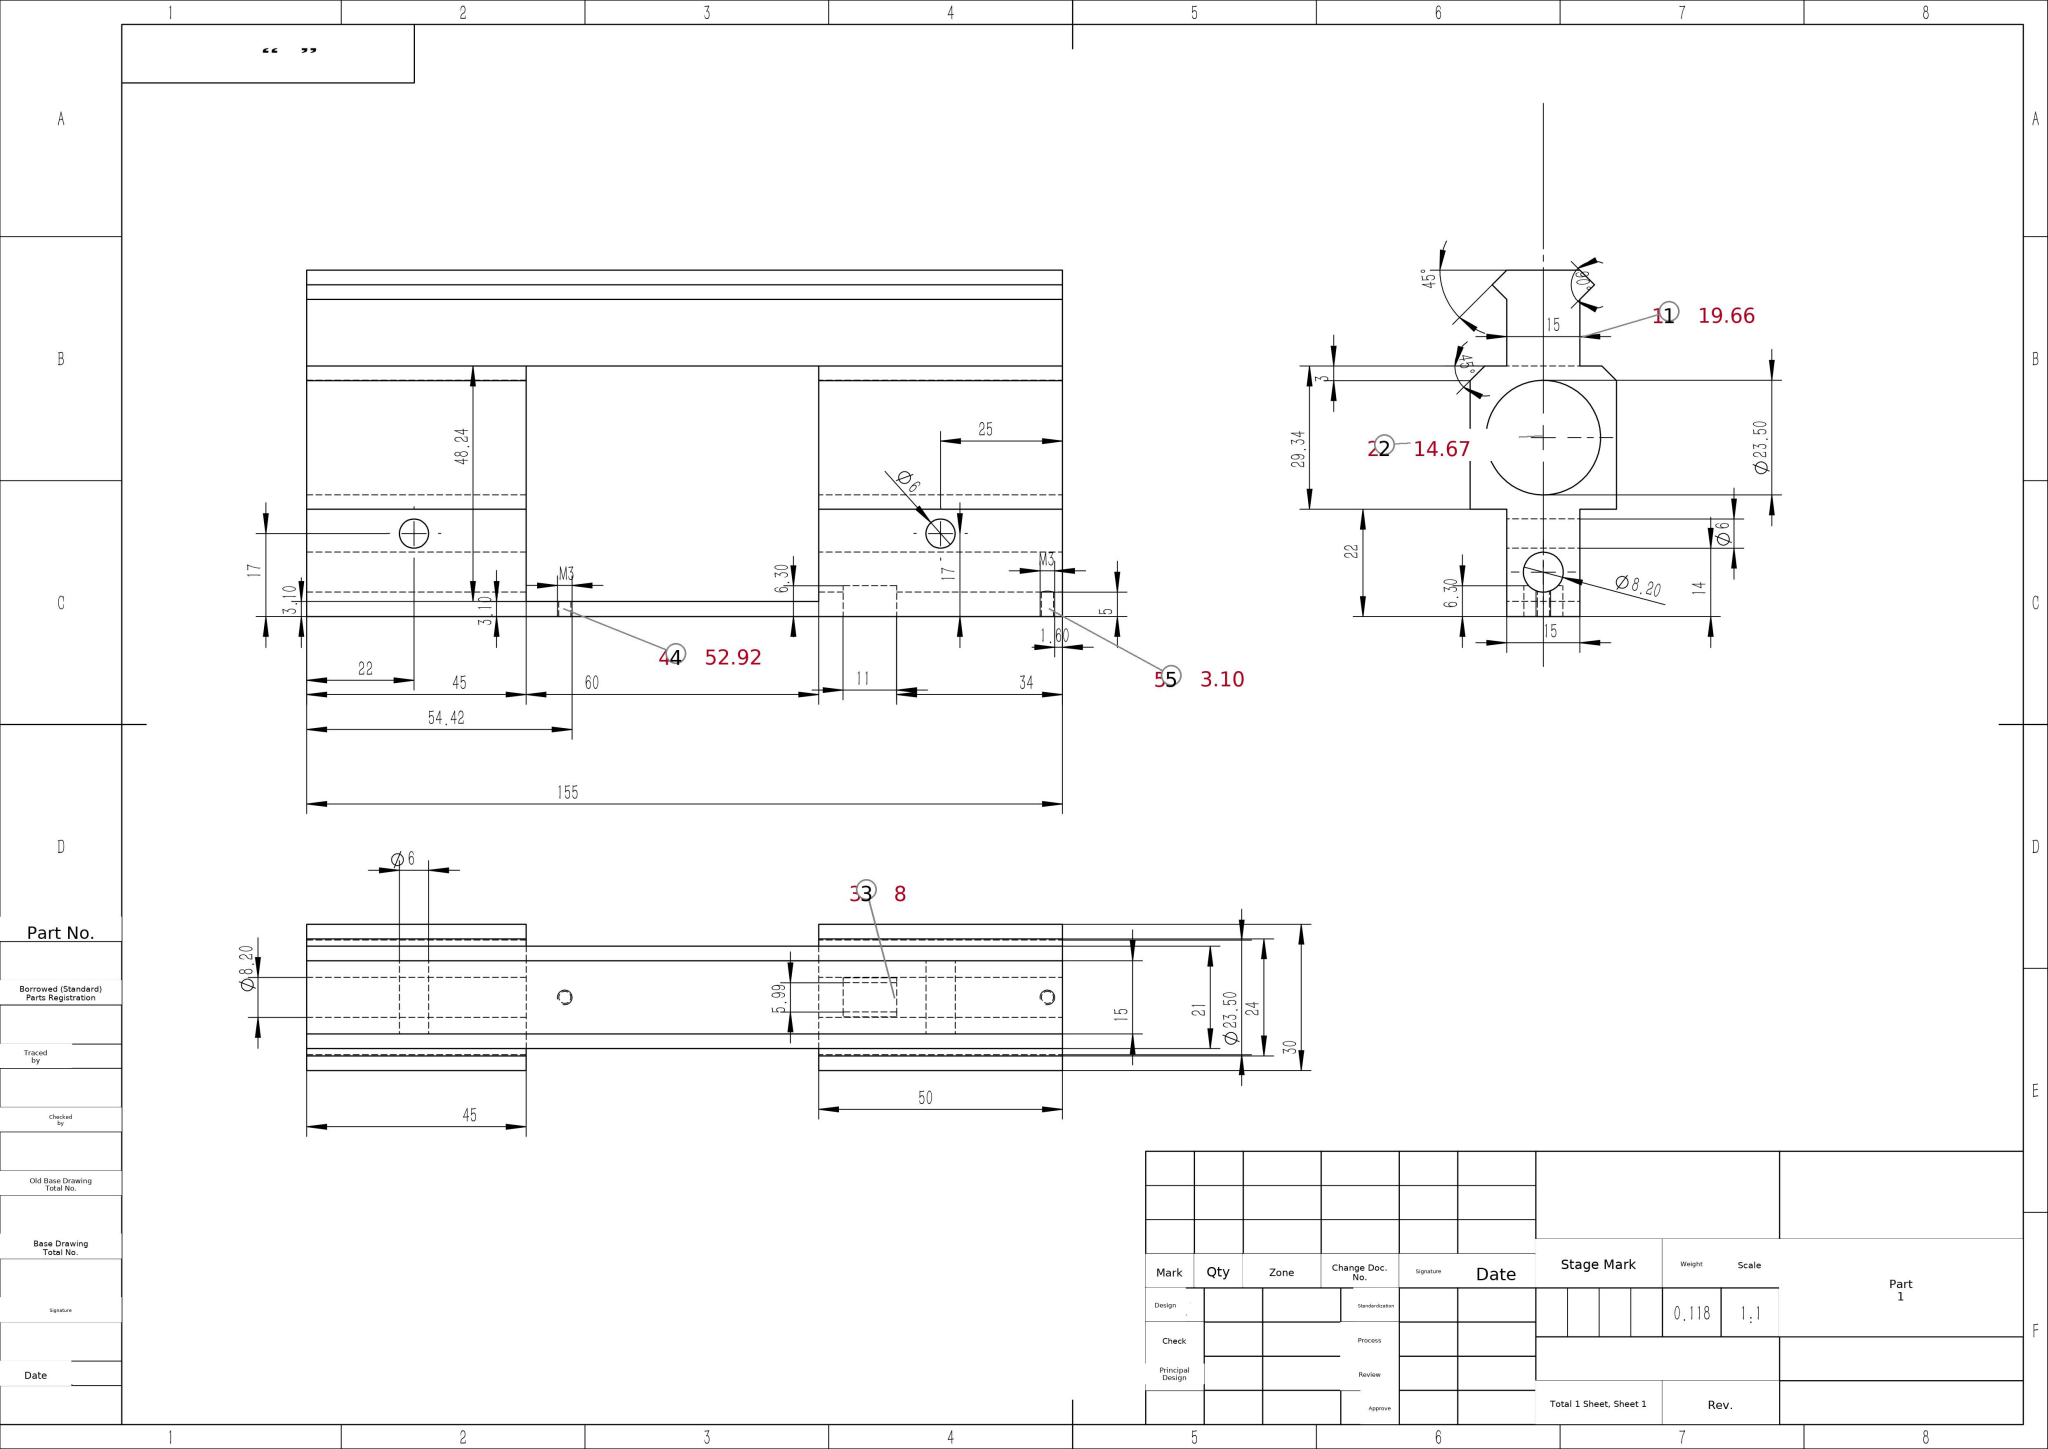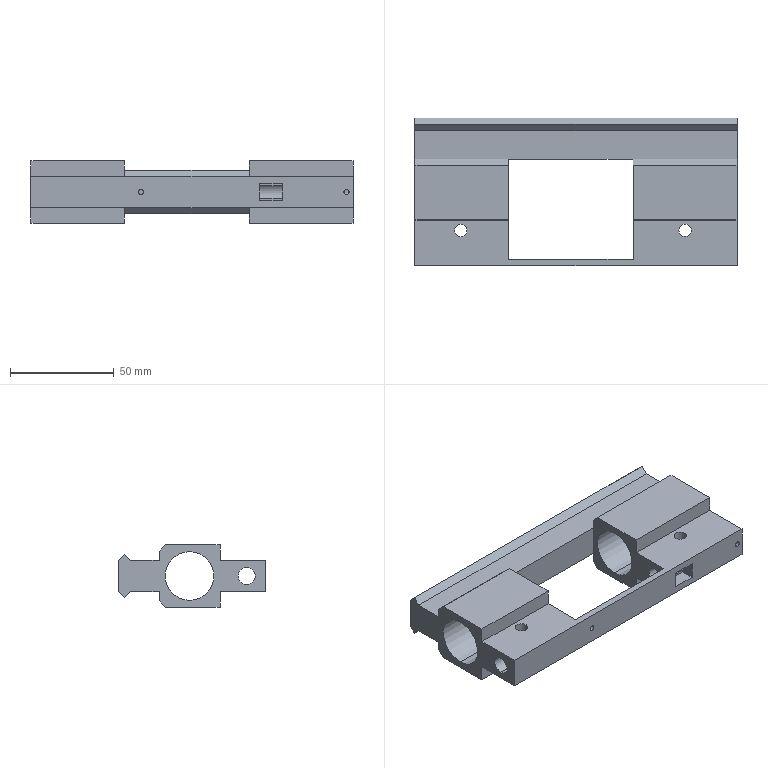Part | SolidWorks | mm | 1 solid | 54 faces | box 155 x 71 x 30 mm | volume 117798 mm3 | plane 38 | cylinder 16 | commonest cylinder face diameters 2.5 x4 6 x4 8.2 x4 23.5 x4
build123d program:
from build123d import *

# Parameters (mm, degrees)
SKETCH1_W              = 15
SKETCH1_H              = 13.66
SKETCH1_W_2            = 30
SKETCH1_H_2            = 29.34
SKETCH1_R              = 11.75
SKETCH1_H_3            = 22
BOSS_EXTRUDE1_DEPTH    = 155
CHAMFER1_SIZE          = 3
SKETCH2_R              = 4.1
CUT_EXTRUDE2_DEPTH     = 155
SKETCH3_R              = 3
CUT_EXTRUDE3_DEPTH     = 77.5
SKETCH4_W              = 60
SKETCH4_H              = 48.24
CUT_EXTRUDE4_DEPTH     = 77.5
M3_TAPPED_HOLE1_REACH  = 173.146
M3_TAPPED_HOLE1_BORE_R = 1.25
SKETCH8_W              = 11
SKETCH8_H              = 6.3
CUT_EXTRUDE6_DEPTH     = 4


with BuildPart() as part:
    # Sketch1 → Boss-Extrude1 (new body)
    # profile 1 of 4: a face of its own
    with BuildSketch(Plane(origin=(0, 0, 0), x_dir=(0, 0, -1), z_dir=(1, 0, 0))):
        Polygon((-7.5, 28.33), (-10.5, 31.33), (-7.5, 34.33), (7.5, 34.33), (10.5, 31.33), (7.5, 28.33), align=None)
    # profile 2 of 4: a face of its own
    with BuildSketch(Plane(origin=(0, 0, 0), x_dir=(0, 0, -1), z_dir=(1, 0, 0))):
        with Locations((0, 21.5)):
            Rectangle(SKETCH1_W, SKETCH1_H)
    # profile 3 of 4: a face of its own
    with BuildSketch(Plane(origin=(0, 0, 0), x_dir=(0, 0, -1), z_dir=(1, 0, 0))):
        Rectangle(SKETCH1_W_2, SKETCH1_H_2)
        Circle(SKETCH1_R, mode=Mode.SUBTRACT)
    # profile 4 of 4: a face of its own
    with BuildSketch(Plane(origin=(0, 0, 0), x_dir=(0, 0, -1), z_dir=(1, 0, 0))):
        with Locations((0, -25.67)):
            Rectangle(SKETCH1_W, SKETCH1_H_3)
    extrude(amount=BOSS_EXTRUDE1_DEPTH)

    # Chamfer1
    chamfer1_edges = [part.edges().sort_by_distance(p)[0] for p in [
        (77.5, 14.67, -15),
        (77.5, 14.67, 15),
    ]]
    chamfer(chamfer1_edges, length=CHAMFER1_SIZE)

    # Sketch2 → Cut-Extrude2 (cut)
    with BuildSketch(Plane(origin=(0, 0, 0), x_dir=(0, 0, -1), z_dir=(1, 0, 0))):
        with Locations((0, -27.57)):
            Circle(SKETCH2_R)
    extrude(amount=CUT_EXTRUDE2_DEPTH, mode=Mode.SUBTRACT)

    # Sketch3 → Cut-Extrude3 (cut, symmetric)
    with BuildSketch(Plane.XY):
        with Locations(Location((22, -19.67, 0), (0, 0, 90))):
            Circle(SKETCH3_R)
        with Locations(Location((130, -19.67, 0), (0, 0, 90))):
            Circle(SKETCH3_R)
    extrude(amount=CUT_EXTRUDE3_DEPTH, both=True, mode=Mode.SUBTRACT)

    # Sketch4 → Cut-Extrude4 (cut, symmetric)
    with BuildSketch(Plane.XY):
        with Locations((75, -9.45)):
            Rectangle(SKETCH4_W, SKETCH4_H)
    extrude(amount=CUT_EXTRUDE4_DEPTH, both=True, mode=Mode.SUBTRACT)

    # M3 Tapped Hole1 bore → M3 Tapped Hole1 (cut, up to next)
    with BuildSketch(Plane(origin=(0, -36.67, 0), x_dir=(-1, 0, 0), z_dir=(0, -1, 0)), mode=Mode.PRIVATE) as m3_tapped_hole1_sk1:
        with Locations((-52.92, 0)):
            Circle(M3_TAPPED_HOLE1_BORE_R)
    m3_tapped_hole1_tool1 = extrude(m3_tapped_hole1_sk1.sketch, amount=-M3_TAPPED_HOLE1_REACH, mode=Mode.PRIVATE) & part.part
    # M3 Tapped Hole1 bore → M3 Tapped Hole1 (cut, up to next)
    with BuildSketch(Plane(origin=(0, -36.67, 0), x_dir=(-1, 0, 0), z_dir=(0, -1, 0)), mode=Mode.PRIVATE) as m3_tapped_hole1_sk2:
        with Locations((-151.9, 0)):
            Circle(M3_TAPPED_HOLE1_BORE_R)
    m3_tapped_hole1_tool2 = extrude(m3_tapped_hole1_sk2.sketch, amount=-M3_TAPPED_HOLE1_REACH, mode=Mode.PRIVATE) & part.part
    add(m3_tapped_hole1_tool1.solids().sort_by_distance((52.92, -36.67, 0))[0], mode=Mode.SUBTRACT)
    add(m3_tapped_hole1_tool2.solids().sort_by_distance((151.9, -36.67, 0))[0], mode=Mode.SUBTRACT)

    # Sketch8 → Cut-Extrude6 (cut, symmetric)
    with BuildSketch(Plane.XY):
        with Locations((115.5, -33.52)):
            Rectangle(SKETCH8_W, SKETCH8_H)
    extrude(amount=CUT_EXTRUDE6_DEPTH, both=True, mode=Mode.SUBTRACT)


solid = part.part